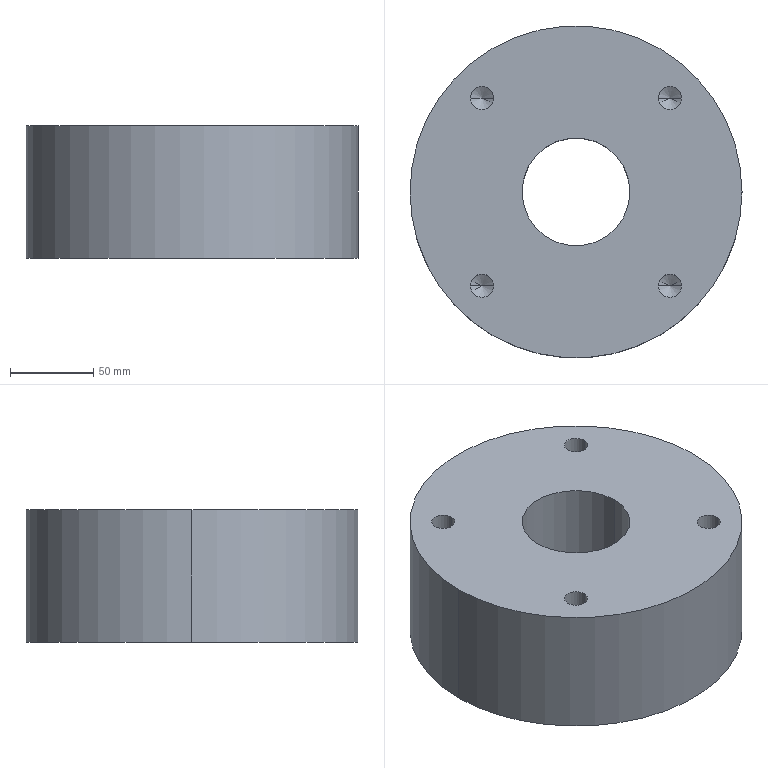Component | SolidWorks | DiePad-1 | 1 solid | 38 faces | box 200 x 200 x 80 mm | volume 2220580 mm3 | cylinder 20 | cone 16 | plane 2 | commonest cylinder face diameters 6.8 x8 14 x8 200 x2 65 x2
build123d program:
from build123d import *

# Parameters (mm, degrees)
SKETCH1_R                  = 100
SKETCH1_R_2                = 32.5
BOSS_EXTRUDE1_DEPTH        = 80
M16_TAPPED_HOLE1_D         = 14
M16_TAPPED_HOLE1_DEPTH     = 38
M16_TAPPED_HOLE1_TIP       = 4.206
M8X1_25_TAPPED_HOLE1_D     = 6.8
M8X1_25_TAPPED_HOLE1_DEPTH = 19.75
M8X1_25_TAPPED_HOLE1_TIP   = 2.043


with BuildPart() as part:
    # Sketch1 → Boss-Extrude1 (new body)
    with BuildSketch(Plane.XY):
        Circle(SKETCH1_R)
        Circle(SKETCH1_R_2, mode=Mode.SUBTRACT)
    extrude(amount=BOSS_EXTRUDE1_DEPTH)

    # M16 Tapped Hole1
    with Locations(Plane.XY.offset(80)):
        with Locations((-56.569, 56.569), (56.569, 56.569), (56.569, -56.569), (-56.569, -56.569)):
            Hole(M16_TAPPED_HOLE1_D / 2, depth=M16_TAPPED_HOLE1_DEPTH)
            with Locations((0, 0, -(M16_TAPPED_HOLE1_DEPTH + M16_TAPPED_HOLE1_TIP / 2))):  # 118° drill point
                Cone(0, M16_TAPPED_HOLE1_D / 2, M16_TAPPED_HOLE1_TIP, mode=Mode.SUBTRACT)

    # M8x1.25 Tapped Hole1
    with Locations(Plane(origin=(0, 0, 0), x_dir=(-1, 0, 0), z_dir=(0, 0, -1))):
        with Locations((-87.5, 0), (0, -87.5), (87.5, 0), (0, 87.5)):
            Hole(M8X1_25_TAPPED_HOLE1_D / 2, depth=M8X1_25_TAPPED_HOLE1_DEPTH)
            with Locations((0, 0, -(M8X1_25_TAPPED_HOLE1_DEPTH + M8X1_25_TAPPED_HOLE1_TIP / 2))):  # 118° drill point
                Cone(0, M8X1_25_TAPPED_HOLE1_D / 2, M8X1_25_TAPPED_HOLE1_TIP, mode=Mode.SUBTRACT)


solid = part.part
STEP:
#1=CARTESIAN_POINT('',(3.579,0.,0.7776));
#2=VERTEX_POINT('',#1);
#3=CARTESIAN_POINT('',(3.311,0.,0.7776));
#4=VERTEX_POINT('',#3);
#5=CARTESIAN_POINT('',(3.445,0.,0.7776));
#6=DIRECTION('',(0.,0.,-1.));
#7=DIRECTION('',(-1.,0.,0.));
#8=AXIS2_PLACEMENT_3D('',#5,#6,#7);
#9=CIRCLE('',#8,0.1339);
#10=EDGE_CURVE('',#2,#4,#9,.T.);
#11=ORIENTED_EDGE('',*,*,#10,.F.);
#12=CARTESIAN_POINT('',(3.579,0.,-0.));
#13=VERTEX_POINT('',#12);
#14=CARTESIAN_POINT('',(3.579,0.,0.));
#15=DIRECTION('',(0.,0.,-1.));
#16=VECTOR('',#15,39.37);
#17=LINE('',#14,#16);
#18=EDGE_CURVE('',#2,#13,#17,.T.);
#19=ORIENTED_EDGE('',*,*,#18,.T.);
#20=CARTESIAN_POINT('',(3.311,0.,-0.));
#21=VERTEX_POINT('',#20);
#22=CARTESIAN_POINT('',(3.445,0.,-0.));
#23=DIRECTION('',(0.,0.,-1.));
#24=DIRECTION('',(-1.,0.,0.));
#25=AXIS2_PLACEMENT_3D('',#22,#23,#24);
#26=CIRCLE('',#25,0.1339);
#27=EDGE_CURVE('',#13,#21,#26,.T.);
#28=ORIENTED_EDGE('',*,*,#27,.T.);
#29=CARTESIAN_POINT('',(3.311,0.,0.));
#30=DIRECTION('',(0.,0.,-1.));
#31=VECTOR('',#30,39.37);
#32=LINE('',#29,#31);
#33=EDGE_CURVE('',#4,#21,#32,.T.);
#34=ORIENTED_EDGE('',*,*,#33,.F.);
#35=EDGE_LOOP('',(#11,#19,#28,#34));
#36=FACE_OUTER_BOUND('',#35,.T.);
#37=CARTESIAN_POINT('',(3.445,0.,0.));
#38=DIRECTION('',(0.,0.,-1.));
#39=DIRECTION('',(-1.,0.,0.));
#40=AXIS2_PLACEMENT_3D('',#37,#38,#39);
#41=CYLINDRICAL_SURFACE('',#40,0.1339);
#42=ADVANCED_FACE('',(#36),#41,.F.);
#43=CARTESIAN_POINT('',(3.445,0.,0.858));
#44=VERTEX_POINT('',#43);
#45=CARTESIAN_POINT('',(3.311,0.,0.7776));
#46=DIRECTION('',(-0.8572,0.,-0.515));
#47=VECTOR('',#46,39.37);
#48=LINE('',#45,#47);
#49=EDGE_CURVE('',#44,#4,#48,.T.);
#50=ORIENTED_EDGE('',*,*,#49,.F.);
#51=CARTESIAN_POINT('',(3.579,0.,0.7776));
#52=DIRECTION('',(0.8572,0.,-0.515));
#53=VECTOR('',#52,39.37);
#54=LINE('',#51,#53);
#55=EDGE_CURVE('',#44,#2,#54,.T.);
#56=ORIENTED_EDGE('',*,*,#55,.T.);
#57=ORIENTED_EDGE('',*,*,#10,.T.);
#58=EDGE_LOOP('',(#50,#56,#57));
#59=FACE_OUTER_BOUND('',#58,.T.);
#60=CARTESIAN_POINT('',(3.445,0.,0.7776));
#61=DIRECTION('',(0.,0.,-1.));
#62=DIRECTION('',(-1.,0.,0.));
#63=AXIS2_PLACEMENT_3D('',#60,#61,#62);
#64=CONICAL_SURFACE('',#63,0.1339,1.03);
#65=ADVANCED_FACE('',(#59),#64,.F.);
#66=CARTESIAN_POINT('',(0.1339,-3.445,0.7776));
#67=VERTEX_POINT('',#66);
#68=CARTESIAN_POINT('',(-0.1339,-3.445,0.7776));
#69=VERTEX_POINT('',#68);
#70=CARTESIAN_POINT('',(0.,-3.445,0.7776));
#71=DIRECTION('',(0.,0.,-1.));
#72=DIRECTION('',(-1.,0.,0.));
#73=AXIS2_PLACEMENT_3D('',#70,#71,#72);
#74=CIRCLE('',#73,0.1339);
#75=EDGE_CURVE('',#67,#69,#74,.T.);
#76=ORIENTED_EDGE('',*,*,#75,.F.);
#77=CARTESIAN_POINT('',(0.1339,-3.445,-0.));
#78=VERTEX_POINT('',#77);
#79=CARTESIAN_POINT('',(0.1339,-3.445,0.));
#80=DIRECTION('',(0.,0.,-1.));
#81=VECTOR('',#80,39.37);
#82=LINE('',#79,#81);
#83=EDGE_CURVE('',#67,#78,#82,.T.);
#84=ORIENTED_EDGE('',*,*,#83,.T.);
#85=CARTESIAN_POINT('',(-0.1339,-3.445,-0.));
#86=VERTEX_POINT('',#85);
#87=CARTESIAN_POINT('',(0.,-3.445,-0.));
#88=DIRECTION('',(0.,0.,-1.));
#89=DIRECTION('',(-1.,0.,0.));
#90=AXIS2_PLACEMENT_3D('',#87,#88,#89);
#91=CIRCLE('',#90,0.1339);
#92=EDGE_CURVE('',#78,#86,#91,.T.);
#93=ORIENTED_EDGE('',*,*,#92,.T.);
#94=CARTESIAN_POINT('',(-0.1339,-3.445,0.));
#95=DIRECTION('',(0.,0.,-1.));
#96=VECTOR('',#95,39.37);
#97=LINE('',#94,#96);
#98=EDGE_CURVE('',#69,#86,#97,.T.);
#99=ORIENTED_EDGE('',*,*,#98,.F.);
#100=EDGE_LOOP('',(#76,#84,#93,#99));
#101=FACE_OUTER_BOUND('',#100,.T.);
#102=CARTESIAN_POINT('',(0.,-3.445,0.));
#103=DIRECTION('',(0.,0.,-1.));
#104=DIRECTION('',(-1.,0.,0.));
#105=AXIS2_PLACEMENT_3D('',#102,#103,#104);
#106=CYLINDRICAL_SURFACE('',#105,0.1339);
#107=ADVANCED_FACE('',(#101),#106,.F.);
#108=CARTESIAN_POINT('',(0.,-3.445,0.858));
#109=VERTEX_POINT('',#108);
#110=CARTESIAN_POINT('',(-0.1339,-3.445,0.7776));
#111=DIRECTION('',(-0.8572,0.,-0.515));
#112=VECTOR('',#111,39.37);
#113=LINE('',#110,#112);
#114=EDGE_CURVE('',#109,#69,#113,.T.);
#115=ORIENTED_EDGE('',*,*,#114,.F.);
#116=CARTESIAN_POINT('',(0.1339,-3.445,0.7776));
#117=DIRECTION('',(0.8572,0.,-0.515));
#118=VECTOR('',#117,39.37);
#119=LINE('',#116,#118);
#120=EDGE_CURVE('',#109,#67,#119,.T.);
#121=ORIENTED_EDGE('',*,*,#120,.T.);
#122=ORIENTED_EDGE('',*,*,#75,.T.);
#123=EDGE_LOOP('',(#115,#121,#122));
#124=FACE_OUTER_BOUND('',#123,.T.);
#125=CARTESIAN_POINT('',(0.,-3.445,0.7776));
#126=DIRECTION('',(0.,0.,-1.));
#127=DIRECTION('',(-1.,0.,0.));
#128=AXIS2_PLACEMENT_3D('',#125,#126,#127);
#129=CONICAL_SURFACE('',#128,0.1339,1.03);
#130=ADVANCED_FACE('',(#124),#129,.F.);
#131=CARTESIAN_POINT('',(-3.311,-0.,0.7776));
#132=VERTEX_POINT('',#131);
#133=CARTESIAN_POINT('',(-3.579,-0.,0.7776));
#134=VERTEX_POINT('',#133);
#135=CARTESIAN_POINT('',(-3.445,-0.,0.7776));
#136=DIRECTION('',(0.,0.,-1.));
#137=DIRECTION('',(-1.,0.,0.));
#138=AXIS2_PLACEMENT_3D('',#135,#136,#137);
#139=CIRCLE('',#138,0.1339);
#140=EDGE_CURVE('',#132,#134,#139,.T.);
#141=ORIENTED_EDGE('',*,*,#140,.F.);
#142=CARTESIAN_POINT('',(-3.311,-0.,-0.));
#143=VERTEX_POINT('',#142);
#144=CARTESIAN_POINT('',(-3.311,-0.,0.));
#145=DIRECTION('',(0.,0.,-1.));
#146=VECTOR('',#145,39.37);
#147=LINE('',#144,#146);
#148=EDGE_CURVE('',#132,#143,#147,.T.);
#149=ORIENTED_EDGE('',*,*,#148,.T.);
#150=CARTESIAN_POINT('',(-3.579,-0.,-0.));
#151=VERTEX_POINT('',#150);
#152=CARTESIAN_POINT('',(-3.445,-0.,-0.));
#153=DIRECTION('',(0.,0.,-1.));
#154=DIRECTION('',(-1.,0.,0.));
#155=AXIS2_PLACEMENT_3D('',#152,#153,#154);
#156=CIRCLE('',#155,0.1339);
#157=EDGE_CURVE('',#143,#151,#156,.T.);
#158=ORIENTED_EDGE('',*,*,#157,.T.);
#159=CARTESIAN_POINT('',(-3.579,-0.,0.));
#160=DIRECTION('',(0.,0.,-1.));
#161=VECTOR('',#160,39.37);
#162=LINE('',#159,#161);
#163=EDGE_CURVE('',#134,#151,#162,.T.);
#164=ORIENTED_EDGE('',*,*,#163,.F.);
#165=EDGE_LOOP('',(#141,#149,#158,#164));
#166=FACE_OUTER_BOUND('',#165,.T.);
#167=CARTESIAN_POINT('',(-3.445,-0.,0.));
#168=DIRECTION('',(0.,0.,-1.));
#169=DIRECTION('',(-1.,0.,0.));
#170=AXIS2_PLACEMENT_3D('',#167,#168,#169);
#171=CYLINDRICAL_SURFACE('',#170,0.1339);
#172=ADVANCED_FACE('',(#166),#171,.F.);
#173=CARTESIAN_POINT('',(-3.445,-0.,0.858));
#174=VERTEX_POINT('',#173);
#175=CARTESIAN_POINT('',(-3.579,-0.,0.7776));
#176=DIRECTION('',(-0.8572,0.,-0.515));
#177=VECTOR('',#176,39.37);
#178=LINE('',#175,#177);
#179=EDGE_CURVE('',#174,#134,#178,.T.);
#180=ORIENTED_EDGE('',*,*,#179,.F.);
#181=CARTESIAN_POINT('',(-3.311,-0.,0.7776));
#182=DIRECTION('',(0.8572,0.,-0.515));
#183=VECTOR('',#182,39.37);
#184=LINE('',#181,#183);
#185=EDGE_CURVE('',#174,#132,#184,.T.);
#186=ORIENTED_EDGE('',*,*,#185,.T.);
#187=ORIENTED_EDGE('',*,*,#140,.T.);
#188=EDGE_LOOP('',(#180,#186,#187));
#189=FACE_OUTER_BOUND('',#188,.T.);
#190=CARTESIAN_POINT('',(-3.445,-0.,0.7776));
#191=DIRECTION('',(0.,0.,-1.));
#192=DIRECTION('',(-1.,0.,0.));
#193=AXIS2_PLACEMENT_3D('',#190,#191,#192);
#194=CONICAL_SURFACE('',#193,0.1339,1.03);
#195=ADVANCED_FACE('',(#189),#194,.F.);
#196=CARTESIAN_POINT('',(0.1339,3.445,0.7776));
#197=VERTEX_POINT('',#196);
#198=CARTESIAN_POINT('',(-0.1339,3.445,0.7776));
#199=VERTEX_POINT('',#198);
#200=CARTESIAN_POINT('',(-0.,3.445,0.7776));
#201=DIRECTION('',(0.,0.,-1.));
#202=DIRECTION('',(-1.,0.,0.));
#203=AXIS2_PLACEMENT_3D('',#200,#201,#202);
#204=CIRCLE('',#203,0.1339);
#205=EDGE_CURVE('',#197,#199,#204,.T.);
#206=ORIENTED_EDGE('',*,*,#205,.F.);
#207=CARTESIAN_POINT('',(0.1339,3.445,-0.));
#208=VERTEX_POINT('',#207);
#209=CARTESIAN_POINT('',(0.1339,3.445,0.));
#210=DIRECTION('',(0.,0.,-1.));
#211=VECTOR('',#210,39.37);
#212=LINE('',#209,#211);
#213=EDGE_CURVE('',#197,#208,#212,.T.);
#214=ORIENTED_EDGE('',*,*,#213,.T.);
#215=CARTESIAN_POINT('',(-0.1339,3.445,-0.));
#216=VERTEX_POINT('',#215);
#217=CARTESIAN_POINT('',(-0.,3.445,-0.));
#218=DIRECTION('',(0.,0.,-1.));
#219=DIRECTION('',(-1.,0.,0.));
#220=AXIS2_PLACEMENT_3D('',#217,#218,#219);
#221=CIRCLE('',#220,0.1339);
#222=EDGE_CURVE('',#208,#216,#221,.T.);
#223=ORIENTED_EDGE('',*,*,#222,.T.);
#224=CARTESIAN_POINT('',(-0.1339,3.445,0.));
#225=DIRECTION('',(0.,0.,-1.));
#226=VECTOR('',#225,39.37);
#227=LINE('',#224,#226);
#228=EDGE_CURVE('',#199,#216,#227,.T.);
#229=ORIENTED_EDGE('',*,*,#228,.F.);
#230=EDGE_LOOP('',(#206,#214,#223,#229));
#231=FACE_OUTER_BOUND('',#230,.T.);
#232=CARTESIAN_POINT('',(-0.,3.445,0.));
#233=DIRECTION('',(0.,0.,-1.));
#234=DIRECTION('',(-1.,0.,0.));
#235=AXIS2_PLACEMENT_3D('',#232,#233,#234);
#236=CYLINDRICAL_SURFACE('',#235,0.1339);
#237=ADVANCED_FACE('',(#231),#236,.F.);
#238=CARTESIAN_POINT('',(-0.,3.445,0.858));
#239=VERTEX_POINT('',#238);
#240=CARTESIAN_POINT('',(-0.1339,3.445,0.7776));
#241=DIRECTION('',(-0.8572,0.,-0.515));
#242=VECTOR('',#241,39.37);
#243=LINE('',#240,#242);
#244=EDGE_CURVE('',#239,#199,#243,.T.);
#245=ORIENTED_EDGE('',*,*,#244,.F.);
#246=CARTESIAN_POINT('',(0.1339,3.445,0.7776));
#247=DIRECTION('',(0.8572,0.,-0.515));
#248=VECTOR('',#247,39.37);
#249=LINE('',#246,#248);
#250=EDGE_CURVE('',#239,#197,#249,.T.);
#251=ORIENTED_EDGE('',*,*,#250,.T.);
#252=ORIENTED_EDGE('',*,*,#205,.T.);
#253=EDGE_LOOP('',(#245,#251,#252));
#254=FACE_OUTER_BOUND('',#253,.T.);
#255=CARTESIAN_POINT('',(-0.,3.445,0.7776));
#256=DIRECTION('',(0.,0.,-1.));
#257=DIRECTION('',(-1.,0.,0.));
#258=AXIS2_PLACEMENT_3D('',#255,#256,#257);
#259=CONICAL_SURFACE('',#258,0.1339,1.03);
#260=ADVANCED_FACE('',(#254),#259,.F.);
#261=CARTESIAN_POINT('',(-2.503,2.227,1.654));
#262=VERTEX_POINT('',#261);
#263=CARTESIAN_POINT('',(-1.952,2.227,1.654));
#264=VERTEX_POINT('',#263);
#265=CARTESIAN_POINT('',(-2.227,2.227,1.654));
#266=DIRECTION('',(0.,0.,1.));
#267=DIRECTION('',(1.,0.,0.));
#268=AXIS2_PLACEMENT_3D('',#265,#266,#267);
#269=CIRCLE('',#268,0.2756);
#270=EDGE_CURVE('',#262,#264,#269,.T.);
#271=ORIENTED_EDGE('',*,*,#270,.F.);
#272=CARTESIAN_POINT('',(-2.503,2.227,3.15));
#273=VERTEX_POINT('',#272);
#274=CARTESIAN_POINT('',(-2.503,2.227,3.15));
#275=DIRECTION('',(0.,0.,1.));
#276=VECTOR('',#275,39.37);
#277=LINE('',#274,#276);
#278=EDGE_CURVE('',#262,#273,#277,.T.);
#279=ORIENTED_EDGE('',*,*,#278,.T.);
#280=CARTESIAN_POINT('',(-1.952,2.227,3.15));
#281=VERTEX_POINT('',#280);
#282=CARTESIAN_POINT('',(-2.227,2.227,3.15));
#283=DIRECTION('',(0.,0.,1.));
#284=DIRECTION('',(1.,0.,0.));
#285=AXIS2_PLACEMENT_3D('',#282,#283,#284);
#286=CIRCLE('',#285,0.2756);
#287=EDGE_CURVE('',#273,#281,#286,.T.);
#288=ORIENTED_EDGE('',*,*,#287,.T.);
#289=CARTESIAN_POINT('',(-1.952,2.227,3.15));
#290=DIRECTION('',(0.,0.,1.));
#291=VECTOR('',#290,39.37);
#292=LINE('',#289,#291);
#293=EDGE_CURVE('',#264,#281,#292,.T.);
#294=ORIENTED_EDGE('',*,*,#293,.F.);
#295=EDGE_LOOP('',(#271,#279,#288,#294));
#296=FACE_OUTER_BOUND('',#295,.T.);
#297=CARTESIAN_POINT('',(-2.227,2.227,3.15));
#298=DIRECTION('',(0.,0.,1.));
#299=DIRECTION('',(1.,0.,0.));
#300=AXIS2_PLACEMENT_3D('',#297,#298,#299);
#301=CYLINDRICAL_SURFACE('',#300,0.2756);
#302=ADVANCED_FACE('',(#296),#301,.F.);
#303=CARTESIAN_POINT('',(-2.227,2.227,1.488));
#304=VERTEX_POINT('',#303);
#305=CARTESIAN_POINT('',(-1.952,2.227,1.654));
#306=DIRECTION('',(0.8572,0.,0.515));
#307=VECTOR('',#306,39.37);
#308=LINE('',#305,#307);
#309=EDGE_CURVE('',#304,#264,#308,.T.);
#310=ORIENTED_EDGE('',*,*,#309,.F.);
#311=CARTESIAN_POINT('',(-2.503,2.227,1.654));
#312=DIRECTION('',(-0.8572,0.,0.515));
#313=VECTOR('',#312,39.37);
#314=LINE('',#311,#313);
#315=EDGE_CURVE('',#304,#262,#314,.T.);
#316=ORIENTED_EDGE('',*,*,#315,.T.);
#317=ORIENTED_EDGE('',*,*,#270,.T.);
#318=EDGE_LOOP('',(#310,#316,#317));
#319=FACE_OUTER_BOUND('',#318,.T.);
#320=CARTESIAN_POINT('',(-2.227,2.227,1.654));
#321=DIRECTION('',(0.,0.,1.));
#322=DIRECTION('',(1.,0.,0.));
#323=AXIS2_PLACEMENT_3D('',#320,#321,#322);
#324=CONICAL_SURFACE('',#323,0.2756,1.03);
#325=ADVANCED_FACE('',(#319),#324,.F.);
#326=CARTESIAN_POINT('',(1.952,2.227,1.654));
#327=VERTEX_POINT('',#326);
#328=CARTESIAN_POINT('',(2.503,2.227,1.654));
#329=VERTEX_POINT('',#328);
#330=CARTESIAN_POINT('',(2.227,2.227,1.654));
#331=DIRECTION('',(0.,0.,1.));
#332=DIRECTION('',(1.,0.,0.));
#333=AXIS2_PLACEMENT_3D('',#330,#331,#332);
#334=CIRCLE('',#333,0.2756);
#335=EDGE_CURVE('',#327,#329,#334,.T.);
#336=ORIENTED_EDGE('',*,*,#335,.F.);
#337=CARTESIAN_POINT('',(1.952,2.227,3.15));
#338=VERTEX_POINT('',#337);
#339=CARTESIAN_POINT('',(1.952,2.227,3.15));
#340=DIRECTION('',(0.,0.,1.));
#341=VECTOR('',#340,39.37);
#342=LINE('',#339,#341);
#343=EDGE_CURVE('',#327,#338,#342,.T.);
#344=ORIENTED_EDGE('',*,*,#343,.T.);
#345=CARTESIAN_POINT('',(2.503,2.227,3.15));
#346=VERTEX_POINT('',#345);
#347=CARTESIAN_POINT('',(2.227,2.227,3.15));
#348=DIRECTION('',(0.,0.,1.));
#349=DIRECTION('',(1.,0.,0.));
#350=AXIS2_PLACEMENT_3D('',#347,#348,#349);
#351=CIRCLE('',#350,0.2756);
#352=EDGE_CURVE('',#338,#346,#351,.T.);
#353=ORIENTED_EDGE('',*,*,#352,.T.);
#354=CARTESIAN_POINT('',(2.503,2.227,3.15));
#355=DIRECTION('',(0.,0.,1.));
#356=VECTOR('',#355,39.37);
#357=LINE('',#354,#356);
#358=EDGE_CURVE('',#329,#346,#357,.T.);
#359=ORIENTED_EDGE('',*,*,#358,.F.);
#360=EDGE_LOOP('',(#336,#344,#353,#359));
#361=FACE_OUTER_BOUND('',#360,.T.);
#362=CARTESIAN_POINT('',(2.227,2.227,3.15));
#363=DIRECTION('',(0.,0.,1.));
#364=DIRECTION('',(1.,0.,0.));
#365=AXIS2_PLACEMENT_3D('',#362,#363,#364);
#366=CYLINDRICAL_SURFACE('',#365,0.2756);
#367=ADVANCED_FACE('',(#361),#366,.F.);
#368=CARTESIAN_POINT('',(2.227,2.227,1.488));
#369=VERTEX_POINT('',#368);
#370=CARTESIAN_POINT('',(2.503,2.227,1.654));
#371=DIRECTION('',(0.8572,0.,0.515));
#372=VECTOR('',#371,39.37);
#373=LINE('',#370,#372);
#374=EDGE_CURVE('',#369,#329,#373,.T.);
#375=ORIENTED_EDGE('',*,*,#374,.F.);
#376=CARTESIAN_POINT('',(1.952,2.227,1.654));
#377=DIRECTION('',(-0.8572,0.,0.515));
#378=VECTOR('',#377,39.37);
#379=LINE('',#376,#378);
#380=EDGE_CURVE('',#369,#327,#379,.T.);
#381=ORIENTED_EDGE('',*,*,#380,.T.);
#382=ORIENTED_EDGE('',*,*,#335,.T.);
#383=EDGE_LOOP('',(#375,#381,#382));
#384=FACE_OUTER_BOUND('',#383,.T.);
#385=CARTESIAN_POINT('',(2.227,2.227,1.654));
#386=DIRECTION('',(0.,0.,1.));
#387=DIRECTION('',(1.,0.,0.));
#388=AXIS2_PLACEMENT_3D('',#385,#386,#387);
#389=CONICAL_SURFACE('',#388,0.2756,1.03);
#390=ADVANCED_FACE('',(#384),#389,.F.);
#391=CARTESIAN_POINT('',(1.952,-2.227,1.654));
#392=VERTEX_POINT('',#391);
#393=CARTESIAN_POINT('',(2.503,-2.227,1.654));
#394=VERTEX_POINT('',#393);
#395=CARTESIAN_POINT('',(2.227,-2.227,1.654));
#396=DIRECTION('',(0.,0.,1.));
#397=DIRECTION('',(1.,0.,0.));
#398=AXIS2_PLACEMENT_3D('',#395,#396,#397);
#399=CIRCLE('',#398,0.2756);
#400=EDGE_CURVE('',#392,#394,#399,.T.);
#401=ORIENTED_EDGE('',*,*,#400,.F.);
#402=CARTESIAN_POINT('',(1.952,-2.227,3.15));
#403=VERTEX_POINT('',#402);
#404=CARTESIAN_POINT('',(1.952,-2.227,3.15));
#405=DIRECTION('',(0.,0.,1.));
#406=VECTOR('',#405,39.37);
#407=LINE('',#404,#406);
#408=EDGE_CURVE('',#392,#403,#407,.T.);
#409=ORIENTED_EDGE('',*,*,#408,.T.);
#410=CARTESIAN_POINT('',(2.503,-2.227,3.15));
#411=VERTEX_POINT('',#410);
#412=CARTESIAN_POINT('',(2.227,-2.227,3.15));
#413=DIRECTION('',(0.,0.,1.));
#414=DIRECTION('',(1.,0.,0.));
#415=AXIS2_PLACEMENT_3D('',#412,#413,#414);
#416=CIRCLE('',#415,0.2756);
#417=EDGE_CURVE('',#403,#411,#416,.T.);
#418=ORIENTED_EDGE('',*,*,#417,.T.);
#419=CARTESIAN_POINT('',(2.503,-2.227,3.15));
#420=DIRECTION('',(0.,0.,1.));
#421=VECTOR('',#420,39.37);
#422=LINE('',#419,#421);
#423=EDGE_CURVE('',#394,#411,#422,.T.);
#424=ORIENTED_EDGE('',*,*,#423,.F.);
#425=EDGE_LOOP('',(#401,#409,#418,#424));
#426=FACE_OUTER_BOUND('',#425,.T.);
#427=CARTESIAN_POINT('',(2.227,-2.227,3.15));
#428=DIRECTION('',(0.,0.,1.));
#429=DIRECTION('',(1.,0.,0.));
#430=AXIS2_PLACEMENT_3D('',#427,#428,#429);
#431=CYLINDRICAL_SURFACE('',#430,0.2756);
#432=ADVANCED_FACE('',(#426),#431,.F.);
#433=CARTESIAN_POINT('',(2.227,-2.227,1.488));
#434=VERTEX_POINT('',#433);
#435=CARTESIAN_POINT('',(2.503,-2.227,1.654));
#436=DIRECTION('',(0.8572,0.,0.515));
#437=VECTOR('',#436,39.37);
#438=LINE('',#435,#437);
#439=EDGE_CURVE('',#434,#394,#438,.T.);
#440=ORIENTED_EDGE('',*,*,#439,.F.);
#441=CARTESIAN_POINT('',(1.952,-2.227,1.654));
#442=DIRECTION('',(-0.8572,0.,0.515));
#443=VECTOR('',#442,39.37);
#444=LINE('',#441,#443);
#445=EDGE_CURVE('',#434,#392,#444,.T.);
#446=ORIENTED_EDGE('',*,*,#445,.T.);
#447=ORIENTED_EDGE('',*,*,#400,.T.);
#448=EDGE_LOOP('',(#440,#446,#447));
#449=FACE_OUTER_BOUND('',#448,.T.);
#450=CARTESIAN_POINT('',(2.227,-2.227,1.654));
#451=DIRECTION('',(0.,0.,1.));
#452=DIRECTION('',(1.,0.,0.));
#453=AXIS2_PLACEMENT_3D('',#450,#451,#452);
#454=CONICAL_SURFACE('',#453,0.2756,1.03);
#455=ADVANCED_FACE('',(#449),#454,.F.);
#456=CARTESIAN_POINT('',(-2.503,-2.227,1.654));
#457=VERTEX_POINT('',#456);
#458=CARTESIAN_POINT('',(-1.952,-2.227,1.654));
#459=VERTEX_POINT('',#458);
#460=CARTESIAN_POINT('',(-2.227,-2.227,1.654));
#461=DIRECTION('',(0.,0.,1.));
#462=DIRECTION('',(1.,0.,0.));
#463=AXIS2_PLACEMENT_3D('',#460,#461,#462);
#464=CIRCLE('',#463,0.2756);
#465=EDGE_CURVE('',#457,#459,#464,.T.);
#466=ORIENTED_EDGE('',*,*,#465,.F.);
#467=CARTESIAN_POINT('',(-2.503,-2.227,3.15));
#468=VERTEX_POINT('',#467);
#469=CARTESIAN_POINT('',(-2.503,-2.227,3.15));
#470=DIRECTION('',(0.,0.,1.));
#471=VECTOR('',#470,39.37);
#472=LINE('',#469,#471);
#473=EDGE_CURVE('',#457,#468,#472,.T.);
#474=ORIENTED_EDGE('',*,*,#473,.T.);
#475=CARTESIAN_POINT('',(-1.952,-2.227,3.15));
#476=VERTEX_POINT('',#475);
#477=CARTESIAN_POINT('',(-2.227,-2.227,3.15));
#478=DIRECTION('',(0.,0.,1.));
#479=DIRECTION('',(1.,0.,0.));
#480=AXIS2_PLACEMENT_3D('',#477,#478,#479);
#481=CIRCLE('',#480,0.2756);
#482=EDGE_CURVE('',#468,#476,#481,.T.);
#483=ORIENTED_EDGE('',*,*,#482,.T.);
#484=CARTESIAN_POINT('',(-1.952,-2.227,3.15));
#485=DIRECTION('',(0.,0.,1.));
#486=VECTOR('',#485,39.37);
#487=LINE('',#484,#486);
#488=EDGE_CURVE('',#459,#476,#487,.T.);
#489=ORIENTED_EDGE('',*,*,#488,.F.);
#490=EDGE_LOOP('',(#466,#474,#483,#489));
#491=FACE_OUTER_BOUND('',#490,.T.);
#492=CARTESIAN_POINT('',(-2.227,-2.227,3.15));
#493=DIRECTION('',(0.,0.,1.));
#494=DIRECTION('',(1.,0.,0.));
#495=AXIS2_PLACEMENT_3D('',#492,#493,#494);
#496=CYLINDRICAL_SURFACE('',#495,0.2756);
#497=ADVANCED_FACE('',(#491),#496,.F.);
#498=CARTESIAN_POINT('',(-2.227,-2.227,1.488));
#499=VERTEX_POINT('',#498);
#500=CARTESIAN_POINT('',(-1.952,-2.227,1.654));
#501=DIRECTION('',(0.8572,0.,0.515));
#502=VECTOR('',#501,39.37);
#503=LINE('',#500,#502);
#504=EDGE_CURVE('',#499,#459,#503,.T.);
#505=ORIENTED_EDGE('',*,*,#504,.F.);
#506=CARTESIAN_POINT('',(-2.503,-2.227,1.654));
#507=DIRECTION('',(-0.8572,0.,0.515));
#508=VECTOR('',#507,39.37);
#509=LINE('',#506,#508);
#510=EDGE_CURVE('',#499,#457,#509,.T.);
#511=ORIENTED_EDGE('',*,*,#510,.T.);
#512=ORIENTED_EDGE('',*,*,#465,.T.);
#513=EDGE_LOOP('',(#505,#511,#512));
#514=FACE_OUTER_BOUND('',#513,.T.);
#515=CARTESIAN_POINT('',(-2.227,-2.227,1.654));
#516=DIRECTION('',(0.,0.,1.));
#517=DIRECTION('',(1.,0.,0.));
#518=AXIS2_PLACEMENT_3D('',#515,#516,#517);
#519=CONICAL_SURFACE('',#518,0.2756,1.03);
#520=ADVANCED_FACE('',(#514),#519,.F.);
#521=CARTESIAN_POINT('',(3.937,0.,3.15));
#522=VERTEX_POINT('',#521);
#523=CARTESIAN_POINT('',(-3.937,0.,3.15));
#524=VERTEX_POINT('',#523);
#525=CARTESIAN_POINT('',(0.,0.,3.15));
#526=DIRECTION('',(0.,0.,1.));
#527=DIRECTION('',(1.,0.,0.));
#528=AXIS2_PLACEMENT_3D('',#525,#526,#527);
#529=CIRCLE('',#528,3.937);
#530=EDGE_CURVE('',#522,#524,#529,.T.);
#531=ORIENTED_EDGE('',*,*,#530,.F.);
#532=CARTESIAN_POINT('',(3.937,0.,0.));
#533=VERTEX_POINT('',#532);
#534=CARTESIAN_POINT('',(3.937,0.,3.15));
#535=DIRECTION('',(0.,0.,-1.));
#536=VECTOR('',#535,39.37);
#537=LINE('',#534,#536);
#538=EDGE_CURVE('',#522,#533,#537,.T.);
#539=ORIENTED_EDGE('',*,*,#538,.T.);
#540=CARTESIAN_POINT('',(-3.937,0.,0.));
#541=VERTEX_POINT('',#540);
#542=CARTESIAN_POINT('',(0.,0.,0.));
#543=DIRECTION('',(0.,0.,1.));
#544=DIRECTION('',(1.,0.,0.));
#545=AXIS2_PLACEMENT_3D('',#542,#543,#544);
#546=CIRCLE('',#545,3.937);
#547=EDGE_CURVE('',#533,#541,#546,.T.);
#548=ORIENTED_EDGE('',*,*,#547,.T.);
#549=CARTESIAN_POINT('',(-3.937,0.,3.15));
#550=DIRECTION('',(0.,0.,-1.));
#551=VECTOR('',#550,39.37);
#552=LINE('',#549,#551);
#553=EDGE_CURVE('',#524,#541,#552,.T.);
#554=ORIENTED_EDGE('',*,*,#553,.F.);
#555=EDGE_LOOP('',(#531,#539,#548,#554));
#556=FACE_OUTER_BOUND('',#555,.T.);
#557=CARTESIAN_POINT('',(0.,0.,3.15));
#558=DIRECTION('',(0.,0.,-1.));
#559=DIRECTION('',(-1.,0.,0.));
#560=AXIS2_PLACEMENT_3D('',#557,#558,#559);
#561=CYLINDRICAL_SURFACE('',#560,3.937);
#562=ADVANCED_FACE('',(#556),#561,.T.);
#563=CARTESIAN_POINT('',(-1.28,0.,3.15));
#564=VERTEX_POINT('',#563);
#565=CARTESIAN_POINT('',(1.28,0.,3.15));
#566=VERTEX_POINT('',#565);
#567=CARTESIAN_POINT('',(0.,0.,3.15));
#568=DIRECTION('',(0.,0.,1.));
#569=DIRECTION('',(1.,0.,0.));
#570=AXIS2_PLACEMENT_3D('',#567,#568,#569);
#571=CIRCLE('',#570,1.28);
#572=EDGE_CURVE('',#564,#566,#571,.T.);
#573=ORIENTED_EDGE('',*,*,#572,.T.);
#574=CARTESIAN_POINT('',(1.28,0.,0.));
#575=VERTEX_POINT('',#574);
#576=CARTESIAN_POINT('',(1.28,0.,3.15));
#577=DIRECTION('',(0.,0.,-1.));
#578=VECTOR('',#577,39.37);
#579=LINE('',#576,#578);
#580=EDGE_CURVE('',#566,#575,#579,.T.);
#581=ORIENTED_EDGE('',*,*,#580,.T.);
#582=CARTESIAN_POINT('',(-1.28,0.,0.));
#583=VERTEX_POINT('',#582);
#584=CARTESIAN_POINT('',(0.,0.,0.));
#585=DIRECTION('',(0.,0.,1.));
#586=DIRECTION('',(1.,0.,0.));
#587=AXIS2_PLACEMENT_3D('',#584,#585,#586);
#588=CIRCLE('',#587,1.28);
#589=EDGE_CURVE('',#583,#575,#588,.T.);
#590=ORIENTED_EDGE('',*,*,#589,.F.);
#591=CARTESIAN_POINT('',(-1.28,0.,3.15));
#592=DIRECTION('',(0.,0.,-1.));
#593=VECTOR('',#592,39.37);
#594=LINE('',#591,#593);
#595=EDGE_CURVE('',#564,#583,#594,.T.);
#596=ORIENTED_EDGE('',*,*,#595,.F.);
#597=EDGE_LOOP('',(#573,#581,#590,#596));
#598=FACE_OUTER_BOUND('',#597,.T.);
#599=CARTESIAN_POINT('',(0.,0.,3.15));
#600=DIRECTION('',(0.,0.,-1.));
#601=DIRECTION('',(-1.,0.,0.));
#602=AXIS2_PLACEMENT_3D('',#599,#600,#601);
#603=CYLINDRICAL_SURFACE('',#602,1.28);
#604=ADVANCED_FACE('',(#598),#603,.F.);
#605=ORIENTED_EDGE('',*,*,#580,.F.);
#606=CARTESIAN_POINT('',(0.,0.,3.15));
#607=DIRECTION('',(0.,0.,1.));
#608=DIRECTION('',(1.,0.,0.));
#609=AXIS2_PLACEMENT_3D('',#606,#607,#608);
#610=CIRCLE('',#609,1.28);
#611=EDGE_CURVE('',#566,#564,#610,.T.);
#612=ORIENTED_EDGE('',*,*,#611,.T.);
#613=ORIENTED_EDGE('',*,*,#595,.T.);
#614=CARTESIAN_POINT('',(0.,0.,0.));
#615=DIRECTION('',(0.,0.,1.));
#616=DIRECTION('',(1.,0.,0.));
#617=AXIS2_PLACEMENT_3D('',#614,#615,#616);
#618=CIRCLE('',#617,1.28);
#619=EDGE_CURVE('',#575,#583,#618,.T.);
#620=ORIENTED_EDGE('',*,*,#619,.F.);
#621=EDGE_LOOP('',(#605,#612,#613,#620));
#622=FACE_OUTER_BOUND('',#621,.T.);
#623=CARTESIAN_POINT('',(0.,0.,3.15));
#624=DIRECTION('',(0.,0.,-1.));
#625=DIRECTION('',(-1.,0.,0.));
#626=AXIS2_PLACEMENT_3D('',#623,#624,#625);
#627=CYLINDRICAL_SURFACE('',#626,1.28);
#628=ADVANCED_FACE('',(#622),#627,.F.);
#629=ORIENTED_EDGE('',*,*,#538,.F.);
#630=CARTESIAN_POINT('',(0.,0.,3.15));
#631=DIRECTION('',(0.,0.,1.));
#632=DIRECTION('',(1.,0.,0.));
#633=AXIS2_PLACEMENT_3D('',#630,#631,#632);
#634=CIRCLE('',#633,3.937);
#635=EDGE_CURVE('',#524,#522,#634,.T.);
#636=ORIENTED_EDGE('',*,*,#635,.F.);
#637=ORIENTED_EDGE('',*,*,#553,.T.);
#638=CARTESIAN_POINT('',(0.,0.,0.));
#639=DIRECTION('',(0.,0.,1.));
#640=DIRECTION('',(1.,0.,0.));
#641=AXIS2_PLACEMENT_3D('',#638,#639,#640);
#642=CIRCLE('',#641,3.937);
#643=EDGE_CURVE('',#541,#533,#642,.T.);
#644=ORIENTED_EDGE('',*,*,#643,.T.);
#645=EDGE_LOOP('',(#629,#636,#637,#644));
#646=FACE_OUTER_BOUND('',#645,.T.);
#647=CARTESIAN_POINT('',(0.,0.,3.15));
#648=DIRECTION('',(0.,0.,-1.));
#649=DIRECTION('',(-1.,0.,0.));
#650=AXIS2_PLACEMENT_3D('',#647,#648,#649);
#651=CYLINDRICAL_SURFACE('',#650,3.937);
#652=ADVANCED_FACE('',(#646),#651,.T.);
#653=CARTESIAN_POINT('',(-2.227,2.227,3.15));
#654=DIRECTION('',(0.,0.,1.));
#655=DIRECTION('',(1.,0.,0.));
#656=AXIS2_PLACEMENT_3D('',#653,#654,#655);
#657=CIRCLE('',#656,0.2756);
#658=EDGE_CURVE('',#281,#273,#657,.T.);
#659=ORIENTED_EDGE('',*,*,#658,.F.);
#660=ORIENTED_EDGE('',*,*,#287,.F.);
#661=EDGE_LOOP('',(#659,#660));
#662=FACE_BOUND('',#661,.T.);
#663=CARTESIAN_POINT('',(2.227,2.227,3.15));
#664=DIRECTION('',(0.,0.,1.));
#665=DIRECTION('',(1.,0.,0.));
#666=AXIS2_PLACEMENT_3D('',#663,#664,#665);
#667=CIRCLE('',#666,0.2756);
#668=EDGE_CURVE('',#346,#338,#667,.T.);
#669=ORIENTED_EDGE('',*,*,#668,.F.);
#670=ORIENTED_EDGE('',*,*,#352,.F.);
#671=EDGE_LOOP('',(#669,#670));
#672=FACE_BOUND('',#671,.T.);
#673=CARTESIAN_POINT('',(2.227,-2.227,3.15));
#674=DIRECTION('',(0.,0.,1.));
#675=DIRECTION('',(1.,0.,0.));
#676=AXIS2_PLACEMENT_3D('',#673,#674,#675);
#677=CIRCLE('',#676,0.2756);
#678=EDGE_CURVE('',#411,#403,#677,.T.);
#679=ORIENTED_EDGE('',*,*,#678,.F.);
#680=ORIENTED_EDGE('',*,*,#417,.F.);
#681=EDGE_LOOP('',(#679,#680));
#682=FACE_BOUND('',#681,.T.);
#683=CARTESIAN_POINT('',(-2.227,-2.227,3.15));
#684=DIRECTION('',(0.,0.,1.));
#685=DIRECTION('',(1.,0.,0.));
#686=AXIS2_PLACEMENT_3D('',#683,#684,#685);
#687=CIRCLE('',#686,0.2756);
#688=EDGE_CURVE('',#476,#468,#687,.T.);
#689=ORIENTED_EDGE('',*,*,#688,.F.);
#690=ORIENTED_EDGE('',*,*,#482,.F.);
#691=EDGE_LOOP('',(#689,#690));
#692=FACE_BOUND('',#691,.T.);
#693=ORIENTED_EDGE('',*,*,#572,.F.);
#694=ORIENTED_EDGE('',*,*,#611,.F.);
#695=EDGE_LOOP('',(#693,#694));
#696=FACE_BOUND('',#695,.T.);
#697=ORIENTED_EDGE('',*,*,#635,.T.);
#698=ORIENTED_EDGE('',*,*,#530,.T.);
#699=EDGE_LOOP('',(#697,#698));
#700=FACE_OUTER_BOUND('',#699,.T.);
#701=CARTESIAN_POINT('',(0.,0.,3.15));
#702=DIRECTION('',(0.,0.,1.));
#703=DIRECTION('',(1.,0.,0.));
#704=AXIS2_PLACEMENT_3D('',#701,#702,#703);
#705=PLANE('',#704);
#706=ADVANCED_FACE('',(#662,#672,#682,#692,#696,#700),#705,.T.);
#707=CARTESIAN_POINT('',(3.445,0.,-0.));
#708=DIRECTION('',(0.,0.,-1.));
#709=DIRECTION('',(-1.,0.,0.));
#710=AXIS2_PLACEMENT_3D('',#707,#708,#709);
#711=CIRCLE('',#710,0.1339);
#712=EDGE_CURVE('',#21,#13,#711,.T.);
#713=ORIENTED_EDGE('',*,*,#712,.F.);
#714=ORIENTED_EDGE('',*,*,#27,.F.);
#715=EDGE_LOOP('',(#713,#714));
#716=FACE_BOUND('',#715,.T.);
#717=CARTESIAN_POINT('',(0.,-3.445,-0.));
#718=DIRECTION('',(0.,0.,-1.));
#719=DIRECTION('',(-1.,0.,0.));
#720=AXIS2_PLACEMENT_3D('',#717,#718,#719);
#721=CIRCLE('',#720,0.1339);
#722=EDGE_CURVE('',#86,#78,#721,.T.);
#723=ORIENTED_EDGE('',*,*,#722,.F.);
#724=ORIENTED_EDGE('',*,*,#92,.F.);
#725=EDGE_LOOP('',(#723,#724));
#726=FACE_BOUND('',#725,.T.);
#727=CARTESIAN_POINT('',(-3.445,-0.,-0.));
#728=DIRECTION('',(0.,0.,-1.));
#729=DIRECTION('',(-1.,0.,0.));
#730=AXIS2_PLACEMENT_3D('',#727,#728,#729);
#731=CIRCLE('',#730,0.1339);
#732=EDGE_CURVE('',#151,#143,#731,.T.);
#733=ORIENTED_EDGE('',*,*,#732,.F.);
#734=ORIENTED_EDGE('',*,*,#157,.F.);
#735=EDGE_LOOP('',(#733,#734));
#736=FACE_BOUND('',#735,.T.);
#737=CARTESIAN_POINT('',(-0.,3.445,-0.));
#738=DIRECTION('',(0.,0.,-1.));
#739=DIRECTION('',(-1.,0.,0.));
#740=AXIS2_PLACEMENT_3D('',#737,#738,#739);
#741=CIRCLE('',#740,0.1339);
#742=EDGE_CURVE('',#216,#208,#741,.T.);
#743=ORIENTED_EDGE('',*,*,#742,.F.);
#744=ORIENTED_EDGE('',*,*,#222,.F.);
#745=EDGE_LOOP('',(#743,#744));
#746=FACE_BOUND('',#745,.T.);
#747=ORIENTED_EDGE('',*,*,#589,.T.);
#748=ORIENTED_EDGE('',*,*,#619,.T.);
#749=EDGE_LOOP('',(#747,#748));
#750=FACE_BOUND('',#749,.T.);
#751=ORIENTED_EDGE('',*,*,#643,.F.);
#752=ORIENTED_EDGE('',*,*,#547,.F.);
#753=EDGE_LOOP('',(#751,#752));
#754=FACE_OUTER_BOUND('',#753,.T.);
#755=CARTESIAN_POINT('',(0.,0.,0.));
#756=DIRECTION('',(0.,0.,1.));
#757=DIRECTION('',(1.,0.,0.));
#758=AXIS2_PLACEMENT_3D('',#755,#756,#757);
#759=PLANE('',#758);
#760=ADVANCED_FACE('',(#716,#726,#736,#746,#750,#754),#759,.F.);
#761=ORIENTED_EDGE('',*,*,#510,.F.);
#762=ORIENTED_EDGE('',*,*,#504,.T.);
#763=CARTESIAN_POINT('',(-2.227,-2.227,1.654));
#764=DIRECTION('',(0.,0.,1.));
#765=DIRECTION('',(1.,0.,0.));
#766=AXIS2_PLACEMENT_3D('',#763,#764,#765);
#767=CIRCLE('',#766,0.2756);
#768=EDGE_CURVE('',#459,#457,#767,.T.);
#769=ORIENTED_EDGE('',*,*,#768,.T.);
#770=EDGE_LOOP('',(#761,#762,#769));
#771=FACE_OUTER_BOUND('',#770,.T.);
#772=CARTESIAN_POINT('',(-2.227,-2.227,1.654));
#773=DIRECTION('',(0.,0.,1.));
#774=DIRECTION('',(1.,0.,0.));
#775=AXIS2_PLACEMENT_3D('',#772,#773,#774);
#776=CONICAL_SURFACE('',#775,0.2756,1.03);
#777=ADVANCED_FACE('',(#771),#776,.F.);
#778=ORIENTED_EDGE('',*,*,#473,.F.);
#779=ORIENTED_EDGE('',*,*,#768,.F.);
#780=ORIENTED_EDGE('',*,*,#488,.T.);
#781=ORIENTED_EDGE('',*,*,#688,.T.);
#782=EDGE_LOOP('',(#778,#779,#780,#781));
#783=FACE_OUTER_BOUND('',#782,.T.);
#784=CARTESIAN_POINT('',(-2.227,-2.227,3.15));
#785=DIRECTION('',(0.,0.,1.));
#786=DIRECTION('',(1.,0.,0.));
#787=AXIS2_PLACEMENT_3D('',#784,#785,#786);
#788=CYLINDRICAL_SURFACE('',#787,0.2756);
#789=ADVANCED_FACE('',(#783),#788,.F.);
#790=ORIENTED_EDGE('',*,*,#445,.F.);
#791=ORIENTED_EDGE('',*,*,#439,.T.);
#792=CARTESIAN_POINT('',(2.227,-2.227,1.654));
#793=DIRECTION('',(0.,0.,1.));
#794=DIRECTION('',(1.,0.,0.));
#795=AXIS2_PLACEMENT_3D('',#792,#793,#794);
#796=CIRCLE('',#795,0.2756);
#797=EDGE_CURVE('',#394,#392,#796,.T.);
#798=ORIENTED_EDGE('',*,*,#797,.T.);
#799=EDGE_LOOP('',(#790,#791,#798));
#800=FACE_OUTER_BOUND('',#799,.T.);
#801=CARTESIAN_POINT('',(2.227,-2.227,1.654));
#802=DIRECTION('',(0.,0.,1.));
#803=DIRECTION('',(1.,0.,0.));
#804=AXIS2_PLACEMENT_3D('',#801,#802,#803);
#805=CONICAL_SURFACE('',#804,0.2756,1.03);
#806=ADVANCED_FACE('',(#800),#805,.F.);
#807=ORIENTED_EDGE('',*,*,#408,.F.);
#808=ORIENTED_EDGE('',*,*,#797,.F.);
#809=ORIENTED_EDGE('',*,*,#423,.T.);
#810=ORIENTED_EDGE('',*,*,#678,.T.);
#811=EDGE_LOOP('',(#807,#808,#809,#810));
#812=FACE_OUTER_BOUND('',#811,.T.);
#813=CARTESIAN_POINT('',(2.227,-2.227,3.15));
#814=DIRECTION('',(0.,0.,1.));
#815=DIRECTION('',(1.,0.,0.));
#816=AXIS2_PLACEMENT_3D('',#813,#814,#815);
#817=CYLINDRICAL_SURFACE('',#816,0.2756);
#818=ADVANCED_FACE('',(#812),#817,.F.);
#819=ORIENTED_EDGE('',*,*,#380,.F.);
#820=ORIENTED_EDGE('',*,*,#374,.T.);
#821=CARTESIAN_POINT('',(2.227,2.227,1.654));
#822=DIRECTION('',(0.,0.,1.));
#823=DIRECTION('',(1.,0.,0.));
#824=AXIS2_PLACEMENT_3D('',#821,#822,#823);
#825=CIRCLE('',#824,0.2756);
#826=EDGE_CURVE('',#329,#327,#825,.T.);
#827=ORIENTED_EDGE('',*,*,#826,.T.);
#828=EDGE_LOOP('',(#819,#820,#827));
#829=FACE_OUTER_BOUND('',#828,.T.);
#830=CARTESIAN_POINT('',(2.227,2.227,1.654));
#831=DIRECTION('',(0.,0.,1.));
#832=DIRECTION('',(1.,0.,0.));
#833=AXIS2_PLACEMENT_3D('',#830,#831,#832);
#834=CONICAL_SURFACE('',#833,0.2756,1.03);
#835=ADVANCED_FACE('',(#829),#834,.F.);
#836=ORIENTED_EDGE('',*,*,#343,.F.);
#837=ORIENTED_EDGE('',*,*,#826,.F.);
#838=ORIENTED_EDGE('',*,*,#358,.T.);
#839=ORIENTED_EDGE('',*,*,#668,.T.);
#840=EDGE_LOOP('',(#836,#837,#838,#839));
#841=FACE_OUTER_BOUND('',#840,.T.);
#842=CARTESIAN_POINT('',(2.227,2.227,3.15));
#843=DIRECTION('',(0.,0.,1.));
#844=DIRECTION('',(1.,0.,0.));
#845=AXIS2_PLACEMENT_3D('',#842,#843,#844);
#846=CYLINDRICAL_SURFACE('',#845,0.2756);
#847=ADVANCED_FACE('',(#841),#846,.F.);
#848=ORIENTED_EDGE('',*,*,#315,.F.);
#849=ORIENTED_EDGE('',*,*,#309,.T.);
#850=CARTESIAN_POINT('',(-2.227,2.227,1.654));
#851=DIRECTION('',(0.,0.,1.));
#852=DIRECTION('',(1.,0.,0.));
#853=AXIS2_PLACEMENT_3D('',#850,#851,#852);
#854=CIRCLE('',#853,0.2756);
#855=EDGE_CURVE('',#264,#262,#854,.T.);
#856=ORIENTED_EDGE('',*,*,#855,.T.);
#857=EDGE_LOOP('',(#848,#849,#856));
#858=FACE_OUTER_BOUND('',#857,.T.);
#859=CARTESIAN_POINT('',(-2.227,2.227,1.654));
#860=DIRECTION('',(0.,0.,1.));
#861=DIRECTION('',(1.,0.,0.));
#862=AXIS2_PLACEMENT_3D('',#859,#860,#861);
#863=CONICAL_SURFACE('',#862,0.2756,1.03);
#864=ADVANCED_FACE('',(#858),#863,.F.);
#865=ORIENTED_EDGE('',*,*,#278,.F.);
#866=ORIENTED_EDGE('',*,*,#855,.F.);
#867=ORIENTED_EDGE('',*,*,#293,.T.);
#868=ORIENTED_EDGE('',*,*,#658,.T.);
#869=EDGE_LOOP('',(#865,#866,#867,#868));
#870=FACE_OUTER_BOUND('',#869,.T.);
#871=CARTESIAN_POINT('',(-2.227,2.227,3.15));
#872=DIRECTION('',(0.,0.,1.));
#873=DIRECTION('',(1.,0.,0.));
#874=AXIS2_PLACEMENT_3D('',#871,#872,#873);
#875=CYLINDRICAL_SURFACE('',#874,0.2756);
#876=ADVANCED_FACE('',(#870),#875,.F.);
#877=ORIENTED_EDGE('',*,*,#250,.F.);
#878=ORIENTED_EDGE('',*,*,#244,.T.);
#879=CARTESIAN_POINT('',(-0.,3.445,0.7776));
#880=DIRECTION('',(0.,0.,-1.));
#881=DIRECTION('',(-1.,0.,0.));
#882=AXIS2_PLACEMENT_3D('',#879,#880,#881);
#883=CIRCLE('',#882,0.1339);
#884=EDGE_CURVE('',#199,#197,#883,.T.);
#885=ORIENTED_EDGE('',*,*,#884,.T.);
#886=EDGE_LOOP('',(#877,#878,#885));
#887=FACE_OUTER_BOUND('',#886,.T.);
#888=CARTESIAN_POINT('',(-0.,3.445,0.7776));
#889=DIRECTION('',(0.,0.,-1.));
#890=DIRECTION('',(-1.,0.,0.));
#891=AXIS2_PLACEMENT_3D('',#888,#889,#890);
#892=CONICAL_SURFACE('',#891,0.1339,1.03);
#893=ADVANCED_FACE('',(#887),#892,.F.);
#894=ORIENTED_EDGE('',*,*,#213,.F.);
#895=ORIENTED_EDGE('',*,*,#884,.F.);
#896=ORIENTED_EDGE('',*,*,#228,.T.);
#897=ORIENTED_EDGE('',*,*,#742,.T.);
#898=EDGE_LOOP('',(#894,#895,#896,#897));
#899=FACE_OUTER_BOUND('',#898,.T.);
#900=CARTESIAN_POINT('',(-0.,3.445,0.));
#901=DIRECTION('',(0.,0.,-1.));
#902=DIRECTION('',(-1.,0.,0.));
#903=AXIS2_PLACEMENT_3D('',#900,#901,#902);
#904=CYLINDRICAL_SURFACE('',#903,0.1339);
#905=ADVANCED_FACE('',(#899),#904,.F.);
#906=ORIENTED_EDGE('',*,*,#185,.F.);
#907=ORIENTED_EDGE('',*,*,#179,.T.);
#908=CARTESIAN_POINT('',(-3.445,-0.,0.7776));
#909=DIRECTION('',(0.,0.,-1.));
#910=DIRECTION('',(-1.,0.,0.));
#911=AXIS2_PLACEMENT_3D('',#908,#909,#910);
#912=CIRCLE('',#911,0.1339);
#913=EDGE_CURVE('',#134,#132,#912,.T.);
#914=ORIENTED_EDGE('',*,*,#913,.T.);
#915=EDGE_LOOP('',(#906,#907,#914));
#916=FACE_OUTER_BOUND('',#915,.T.);
#917=CARTESIAN_POINT('',(-3.445,-0.,0.7776));
#918=DIRECTION('',(0.,0.,-1.));
#919=DIRECTION('',(-1.,0.,0.));
#920=AXIS2_PLACEMENT_3D('',#917,#918,#919);
#921=CONICAL_SURFACE('',#920,0.1339,1.03);
#922=ADVANCED_FACE('',(#916),#921,.F.);
#923=ORIENTED_EDGE('',*,*,#148,.F.);
#924=ORIENTED_EDGE('',*,*,#913,.F.);
#925=ORIENTED_EDGE('',*,*,#163,.T.);
#926=ORIENTED_EDGE('',*,*,#732,.T.);
#927=EDGE_LOOP('',(#923,#924,#925,#926));
#928=FACE_OUTER_BOUND('',#927,.T.);
#929=CARTESIAN_POINT('',(-3.445,-0.,0.));
#930=DIRECTION('',(0.,0.,-1.));
#931=DIRECTION('',(-1.,0.,0.));
#932=AXIS2_PLACEMENT_3D('',#929,#930,#931);
#933=CYLINDRICAL_SURFACE('',#932,0.1339);
#934=ADVANCED_FACE('',(#928),#933,.F.);
#935=ORIENTED_EDGE('',*,*,#120,.F.);
#936=ORIENTED_EDGE('',*,*,#114,.T.);
#937=CARTESIAN_POINT('',(0.,-3.445,0.7776));
#938=DIRECTION('',(0.,0.,-1.));
#939=DIRECTION('',(-1.,0.,0.));
#940=AXIS2_PLACEMENT_3D('',#937,#938,#939);
#941=CIRCLE('',#940,0.1339);
#942=EDGE_CURVE('',#69,#67,#941,.T.);
#943=ORIENTED_EDGE('',*,*,#942,.T.);
#944=EDGE_LOOP('',(#935,#936,#943));
#945=FACE_OUTER_BOUND('',#944,.T.);
#946=CARTESIAN_POINT('',(0.,-3.445,0.7776));
#947=DIRECTION('',(0.,0.,-1.));
#948=DIRECTION('',(-1.,0.,0.));
#949=AXIS2_PLACEMENT_3D('',#946,#947,#948);
#950=CONICAL_SURFACE('',#949,0.1339,1.03);
#951=ADVANCED_FACE('',(#945),#950,.F.);
#952=ORIENTED_EDGE('',*,*,#83,.F.);
#953=ORIENTED_EDGE('',*,*,#942,.F.);
#954=ORIENTED_EDGE('',*,*,#98,.T.);
#955=ORIENTED_EDGE('',*,*,#722,.T.);
#956=EDGE_LOOP('',(#952,#953,#954,#955));
#957=FACE_OUTER_BOUND('',#956,.T.);
#958=CARTESIAN_POINT('',(0.,-3.445,0.));
#959=DIRECTION('',(0.,0.,-1.));
#960=DIRECTION('',(-1.,0.,0.));
#961=AXIS2_PLACEMENT_3D('',#958,#959,#960);
#962=CYLINDRICAL_SURFACE('',#961,0.1339);
#963=ADVANCED_FACE('',(#957),#962,.F.);
#964=ORIENTED_EDGE('',*,*,#55,.F.);
#965=ORIENTED_EDGE('',*,*,#49,.T.);
#966=CARTESIAN_POINT('',(3.445,0.,0.7776));
#967=DIRECTION('',(0.,0.,-1.));
#968=DIRECTION('',(-1.,0.,0.));
#969=AXIS2_PLACEMENT_3D('',#966,#967,#968);
#970=CIRCLE('',#969,0.1339);
#971=EDGE_CURVE('',#4,#2,#970,.T.);
#972=ORIENTED_EDGE('',*,*,#971,.T.);
#973=EDGE_LOOP('',(#964,#965,#972));
#974=FACE_OUTER_BOUND('',#973,.T.);
#975=CARTESIAN_POINT('',(3.445,0.,0.7776));
#976=DIRECTION('',(0.,0.,-1.));
#977=DIRECTION('',(-1.,0.,0.));
#978=AXIS2_PLACEMENT_3D('',#975,#976,#977);
#979=CONICAL_SURFACE('',#978,0.1339,1.03);
#980=ADVANCED_FACE('',(#974),#979,.F.);
#981=ORIENTED_EDGE('',*,*,#18,.F.);
#982=ORIENTED_EDGE('',*,*,#971,.F.);
#983=ORIENTED_EDGE('',*,*,#33,.T.);
#984=ORIENTED_EDGE('',*,*,#712,.T.);
#985=EDGE_LOOP('',(#981,#982,#983,#984));
#986=FACE_OUTER_BOUND('',#985,.T.);
#987=CARTESIAN_POINT('',(3.445,0.,0.));
#988=DIRECTION('',(0.,0.,-1.));
#989=DIRECTION('',(-1.,0.,0.));
#990=AXIS2_PLACEMENT_3D('',#987,#988,#989);
#991=CYLINDRICAL_SURFACE('',#990,0.1339);
#992=ADVANCED_FACE('',(#986),#991,.F.);
#993=CLOSED_SHELL('',(#42,#65,#107,#130,#172,#195,#237,#260,#302,#325,#367,#390,#432,#455,#497,#520,#562,#604,#628,#652,#706,#760,#777,#789,#806,#818,#835,#847,#864,#876,#893,#905,#922,#934,#951,#963,#980,#992));
#994=MANIFOLD_SOLID_BREP('',#993);
#995=CARTESIAN_POINT('',(0.,0.,0.));
#996=DIRECTION('',(0.,0.,1.));
#997=DIRECTION('',(1.,0.,0.));
#998=AXIS2_PLACEMENT_3D('',#995,#996,#997);
#999=(LENGTH_UNIT()NAMED_UNIT(*)SI_UNIT($,.METRE.));
#1000=LENGTH_MEASURE_WITH_UNIT(LENGTH_MEASURE(0.0254),#999);
#1001=DIMENSIONAL_EXPONENTS(1.,0.,0.,0.,0.,0.,0.);
#1002=(CONVERSION_BASED_UNIT('',#1000)LENGTH_UNIT()NAMED_UNIT(#1001));
#1003=UNCERTAINTY_MEASURE_WITH_UNIT(LENGTH_MEASURE(0.00001),#1002,'','');
#1004=(NAMED_UNIT(*)PLANE_ANGLE_UNIT()SI_UNIT($,.RADIAN.));
#1005=(NAMED_UNIT(*)SI_UNIT($,.STERADIAN.)SOLID_ANGLE_UNIT());
#1006=(GEOMETRIC_REPRESENTATION_CONTEXT(3)GLOBAL_UNCERTAINTY_ASSIGNED_CONTEXT((#1003))GLOBAL_UNIT_ASSIGNED_CONTEXT((#1002,#1004,#1005))REPRESENTATION_CONTEXT('',''));
#1007=ADVANCED_BREP_SHAPE_REPRESENTATION('',(#994,#998),#1006);
#1008=COLOUR_RGB('',0.7922,0.8196,0.9333);
#1009=FILL_AREA_STYLE_COLOUR('',#1008);
#1010=FILL_AREA_STYLE('',(#1009));
#1011=SURFACE_STYLE_FILL_AREA(#1010);
#1012=SURFACE_SIDE_STYLE('',(#1011));
#1013=SURFACE_STYLE_USAGE(.BOTH.,#1012);
#1014=PRESENTATION_STYLE_ASSIGNMENT((#1013));
#1015=STYLED_ITEM('',(#1014),#994);
#1016=PRESENTATION_LAYER_ASSIGNMENT('','',(#1015));
#1017=(LENGTH_UNIT()NAMED_UNIT(*)SI_UNIT($,.METRE.));
#1018=LENGTH_MEASURE_WITH_UNIT(LENGTH_MEASURE(0.0254),#1017);
#1019=DIMENSIONAL_EXPONENTS(1.,0.,0.,0.,0.,0.,0.);
#1020=(CONVERSION_BASED_UNIT('',#1018)LENGTH_UNIT()NAMED_UNIT(#1019));
#1021=UNCERTAINTY_MEASURE_WITH_UNIT(LENGTH_MEASURE(0.00001),#1020,'','');
#1022=(NAMED_UNIT(*)PLANE_ANGLE_UNIT()SI_UNIT($,.RADIAN.));
#1023=(NAMED_UNIT(*)SI_UNIT($,.STERADIAN.)SOLID_ANGLE_UNIT());
#1024=(GEOMETRIC_REPRESENTATION_CONTEXT(3)GLOBAL_UNCERTAINTY_ASSIGNED_CONTEXT((#1021))GLOBAL_UNIT_ASSIGNED_CONTEXT((#1020,#1022,#1023))REPRESENTATION_CONTEXT('',''));
#1025=MECHANICAL_DESIGN_GEOMETRIC_PRESENTATION_REPRESENTATION('',(#1015),#1024);